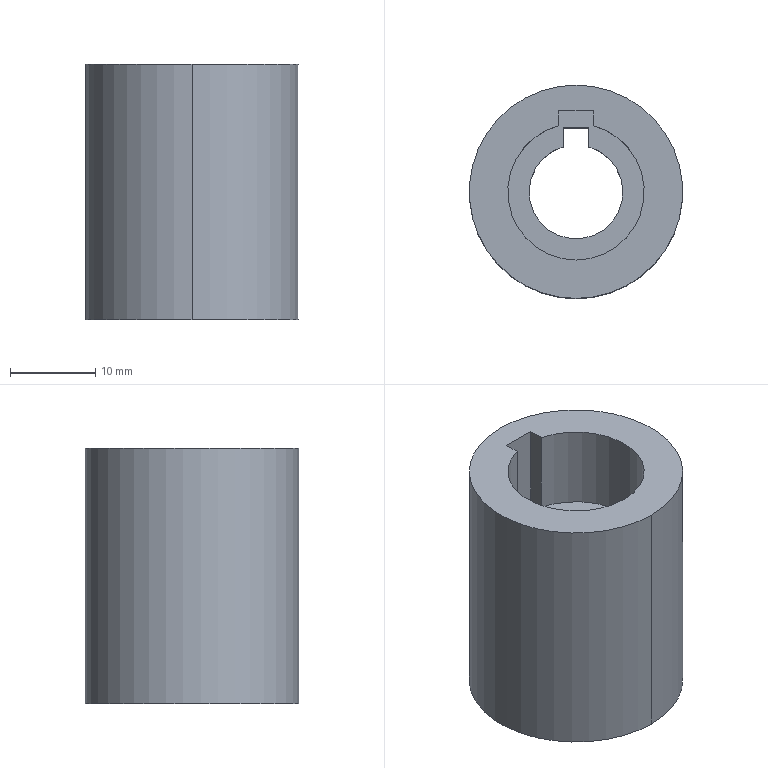Component | SolidWorks | Coupling-1 | 1 solid | 14 faces | box 25 x 25 x 30 mm | volume 10627 mm3 | plane 9 | cylinder 5 | commonest cylinder face diameters 16 x2 25 x2 11 x1
build123d program:
from build123d import *

# Parameters (mm, degrees)
SKETCH1_R               = 12.5
BOSS_EXTRUDE1_DEPTH     = 30
CUT_EXTRUDE1_DEPTH      = 35.821
CUT_EXTRUDE1_DEPTH_BACK = 35.821
SKETCH2_R               = 5
SKETCH3_R               = 8
CUT_EXTRUDE2_DEPTH      = 10
SKETCH4_R               = 5.5
CUT_EXTRUDE3_DEPTH      = 20
SKETCH5_W               = 3
SKETCH5_H               = 4
CUT_EXTRUDE4_DEPTH      = 20
SKETCH6_W               = 4
SKETCH6_H               = 3
CUT_EXTRUDE5_DEPTH      = 10


with BuildPart() as part:
    # Sketch1 → Boss-Extrude1 (new body)
    with BuildSketch(Plane(origin=(0, 0, 0), x_dir=(1, 0, 0), z_dir=(0, 1, 0))):
        with Locations(Location((0, 0, 0), (0, 0, 270))):
            Circle(SKETCH1_R)
    extrude(amount=BOSS_EXTRUDE1_DEPTH)

    # Sketch2 → Cut-Extrude1 (cut, two sides: drawn at the far end of the back side and taken through both)
    with BuildSketch(Plane(origin=(0, 30, 0), x_dir=(1, 0, 0), z_dir=(0, 1, 0)).offset(-CUT_EXTRUDE1_DEPTH_BACK)):
        with Locations(Location((0, 0, 0), (0, 0, 270))):
            Circle(SKETCH2_R)
    extrude(amount=CUT_EXTRUDE1_DEPTH + CUT_EXTRUDE1_DEPTH_BACK, mode=Mode.SUBTRACT)

    # Sketch3 → Cut-Extrude2 (cut)
    with BuildSketch(Plane(origin=(0, 30, 0), x_dir=(1, 0, 0), z_dir=(0, 1, 0))):
        with Locations(Location((0, 0, 0), (0, 0, 270))):
            Circle(SKETCH3_R)
    extrude(amount=-CUT_EXTRUDE2_DEPTH, mode=Mode.SUBTRACT)

    # Sketch4 → Cut-Extrude3 (cut)
    with BuildSketch(Plane.XZ):
        with Locations(Location((0, 0, 0), (0, 0, 270))):
            Circle(SKETCH4_R)
    extrude(amount=-CUT_EXTRUDE3_DEPTH, mode=Mode.SUBTRACT)

    # Sketch5 → Cut-Extrude4 (cut)
    with BuildSketch(Plane.XZ):
        with Locations((0, -5.5)):
            Rectangle(SKETCH5_W, SKETCH5_H)
    extrude(amount=-CUT_EXTRUDE4_DEPTH, mode=Mode.SUBTRACT)

    # Sketch6 → Cut-Extrude5 (cut)
    with BuildSketch(Plane(origin=(0, 30, 0), x_dir=(1, 0, 0), z_dir=(0, 1, 0))):
        with Locations((0, 8)):
            Rectangle(SKETCH6_W, SKETCH6_H)
    extrude(amount=-CUT_EXTRUDE5_DEPTH, mode=Mode.SUBTRACT)


solid = part.part

# Placed as in the assembly
solid = solid.moved(Location((0, -208.707, -673.144), (90, 0, 0)))
STEP:
#1=COLOUR_RGB('',0.7922,0.8196,0.9333);
#2=FILL_AREA_STYLE_COLOUR('',#1);
#3=FILL_AREA_STYLE('',(#2));
#4=SURFACE_STYLE_FILL_AREA(#3);
#5=SURFACE_SIDE_STYLE('',(#4));
#6=SURFACE_STYLE_USAGE(.BOTH.,#5);
#7=PRESENTATION_STYLE_ASSIGNMENT((#6));
#8=CARTESIAN_POINT('',(0.,-8.532,-25.714));
#9=VERTEX_POINT('',#8);
#10=CARTESIAN_POINT('',(0.07874,-7.912,-25.714));
#11=VERTEX_POINT('',#10);
#12=CARTESIAN_POINT('',(-0.,-8.217,-25.714));
#13=DIRECTION('',(0.,0.,1.));
#14=DIRECTION('',(0.,-1.,0.));
#15=AXIS2_PLACEMENT_3D('',#12,#13,#14);
#16=CIRCLE('',#15,0.315);
#17=EDGE_CURVE('',#9,#11,#16,.T.);
#18=ORIENTED_EDGE('',*,*,#17,.F.);
#19=CARTESIAN_POINT('',(0.,-8.532,-25.321));
#20=VERTEX_POINT('',#19);
#21=CARTESIAN_POINT('',(0.,-8.532,-25.714));
#22=DIRECTION('',(0.,0.,1.));
#23=VECTOR('',#22,39.37);
#24=LINE('',#21,#23);
#25=EDGE_CURVE('',#9,#20,#24,.T.);
#26=ORIENTED_EDGE('',*,*,#25,.T.);
#27=CARTESIAN_POINT('',(0.07874,-7.912,-25.321));
#28=VERTEX_POINT('',#27);
#29=CARTESIAN_POINT('',(-0.,-8.217,-25.321));
#30=DIRECTION('',(0.,0.,1.));
#31=DIRECTION('',(0.,-1.,0.));
#32=AXIS2_PLACEMENT_3D('',#29,#30,#31);
#33=CIRCLE('',#32,0.315);
#34=EDGE_CURVE('',#20,#28,#33,.T.);
#35=ORIENTED_EDGE('',*,*,#34,.T.);
#36=CARTESIAN_POINT('',(0.07874,-7.912,-25.714));
#37=DIRECTION('',(-0.,-0.,-1.));
#38=VECTOR('',#37,39.37);
#39=LINE('',#36,#38);
#40=EDGE_CURVE('',#28,#11,#39,.T.);
#41=ORIENTED_EDGE('',*,*,#40,.T.);
#42=EDGE_LOOP('',(#18,#26,#35,#41));
#43=FACE_OUTER_BOUND('',#42,.T.);
#44=CARTESIAN_POINT('',(-0.,-8.217,-25.714));
#45=DIRECTION('',(0.,0.,1.));
#46=DIRECTION('',(0.,-1.,0.));
#47=AXIS2_PLACEMENT_3D('',#44,#45,#46);
#48=CYLINDRICAL_SURFACE('',#47,0.315);
#49=ADVANCED_FACE('',(#43),#48,.F.);
#50=CARTESIAN_POINT('',(0.,-8.709,-25.321));
#51=VERTEX_POINT('',#50);
#52=CARTESIAN_POINT('',(-0.,-7.725,-25.321));
#53=VERTEX_POINT('',#52);
#54=CARTESIAN_POINT('',(-0.,-8.217,-25.321));
#55=DIRECTION('',(0.,0.,1.));
#56=DIRECTION('',(0.,-1.,0.));
#57=AXIS2_PLACEMENT_3D('',#54,#55,#56);
#58=CIRCLE('',#57,0.4921);
#59=EDGE_CURVE('',#51,#53,#58,.T.);
#60=ORIENTED_EDGE('',*,*,#59,.F.);
#61=CARTESIAN_POINT('',(0.,-8.709,-26.502));
#62=VERTEX_POINT('',#61);
#63=CARTESIAN_POINT('',(0.,-8.709,-25.321));
#64=DIRECTION('',(-0.,-0.,-1.));
#65=VECTOR('',#64,39.37);
#66=LINE('',#63,#65);
#67=EDGE_CURVE('',#51,#62,#66,.T.);
#68=ORIENTED_EDGE('',*,*,#67,.T.);
#69=CARTESIAN_POINT('',(-0.,-7.725,-26.502));
#70=VERTEX_POINT('',#69);
#71=CARTESIAN_POINT('',(-0.,-8.217,-26.502));
#72=DIRECTION('',(0.,0.,1.));
#73=DIRECTION('',(0.,-1.,0.));
#74=AXIS2_PLACEMENT_3D('',#71,#72,#73);
#75=CIRCLE('',#74,0.4921);
#76=EDGE_CURVE('',#62,#70,#75,.T.);
#77=ORIENTED_EDGE('',*,*,#76,.T.);
#78=CARTESIAN_POINT('',(-0.,-7.725,-25.321));
#79=DIRECTION('',(-0.,-0.,-1.));
#80=VECTOR('',#79,39.37);
#81=LINE('',#78,#80);
#82=EDGE_CURVE('',#53,#70,#81,.T.);
#83=ORIENTED_EDGE('',*,*,#82,.F.);
#84=EDGE_LOOP('',(#60,#68,#77,#83));
#85=FACE_OUTER_BOUND('',#84,.T.);
#86=CARTESIAN_POINT('',(-0.,-8.217,-25.321));
#87=DIRECTION('',(-0.,-0.,-1.));
#88=DIRECTION('',(-0.,1.,0.));
#89=AXIS2_PLACEMENT_3D('',#86,#87,#88);
#90=CYLINDRICAL_SURFACE('',#89,0.4921);
#91=ADVANCED_FACE('',(#85),#90,.T.);
#92=ORIENTED_EDGE('',*,*,#67,.F.);
#93=CARTESIAN_POINT('',(-0.,-8.217,-25.321));
#94=DIRECTION('',(0.,0.,1.));
#95=DIRECTION('',(0.,-1.,0.));
#96=AXIS2_PLACEMENT_3D('',#93,#94,#95);
#97=CIRCLE('',#96,0.4921);
#98=EDGE_CURVE('',#53,#51,#97,.T.);
#99=ORIENTED_EDGE('',*,*,#98,.F.);
#100=ORIENTED_EDGE('',*,*,#82,.T.);
#101=CARTESIAN_POINT('',(-0.,-8.217,-26.502));
#102=DIRECTION('',(0.,0.,1.));
#103=DIRECTION('',(0.,-1.,0.));
#104=AXIS2_PLACEMENT_3D('',#101,#102,#103);
#105=CIRCLE('',#104,0.4921);
#106=EDGE_CURVE('',#70,#62,#105,.T.);
#107=ORIENTED_EDGE('',*,*,#106,.T.);
#108=EDGE_LOOP('',(#92,#99,#100,#107));
#109=FACE_OUTER_BOUND('',#108,.T.);
#110=CARTESIAN_POINT('',(-0.,-8.217,-25.321));
#111=DIRECTION('',(-0.,-0.,-1.));
#112=DIRECTION('',(-0.,1.,0.));
#113=AXIS2_PLACEMENT_3D('',#110,#111,#112);
#114=CYLINDRICAL_SURFACE('',#113,0.4921);
#115=ADVANCED_FACE('',(#109),#114,.T.);
#116=CARTESIAN_POINT('',(0.07874,-7.843,-25.321));
#117=VERTEX_POINT('',#116);
#118=CARTESIAN_POINT('',(0.07874,-7.961,-25.321));
#119=DIRECTION('',(-0.,1.,-0.));
#120=VECTOR('',#119,39.37);
#121=LINE('',#118,#120);
#122=EDGE_CURVE('',#28,#117,#121,.T.);
#123=ORIENTED_EDGE('',*,*,#122,.F.);
#124=ORIENTED_EDGE('',*,*,#34,.F.);
#125=CARTESIAN_POINT('',(-0.07874,-7.912,-25.321));
#126=VERTEX_POINT('',#125);
#127=CARTESIAN_POINT('',(-0.,-8.217,-25.321));
#128=DIRECTION('',(0.,0.,1.));
#129=DIRECTION('',(0.,-1.,0.));
#130=AXIS2_PLACEMENT_3D('',#127,#128,#129);
#131=CIRCLE('',#130,0.315);
#132=EDGE_CURVE('',#126,#20,#131,.T.);
#133=ORIENTED_EDGE('',*,*,#132,.F.);
#134=CARTESIAN_POINT('',(-0.07874,-7.843,-25.321));
#135=VERTEX_POINT('',#134);
#136=CARTESIAN_POINT('',(-0.07874,-7.961,-25.321));
#137=DIRECTION('',(0.,-1.,0.));
#138=VECTOR('',#137,39.37);
#139=LINE('',#136,#138);
#140=EDGE_CURVE('',#135,#126,#139,.T.);
#141=ORIENTED_EDGE('',*,*,#140,.F.);
#142=CARTESIAN_POINT('',(-0.07874,-7.843,-25.321));
#143=DIRECTION('',(-1.,-0.,0.));
#144=VECTOR('',#143,39.37);
#145=LINE('',#142,#144);
#146=EDGE_CURVE('',#117,#135,#145,.T.);
#147=ORIENTED_EDGE('',*,*,#146,.F.);
#148=EDGE_LOOP('',(#123,#124,#133,#141,#147));
#149=FACE_BOUND('',#148,.T.);
#150=ORIENTED_EDGE('',*,*,#98,.T.);
#151=ORIENTED_EDGE('',*,*,#59,.T.);
#152=EDGE_LOOP('',(#150,#151));
#153=FACE_OUTER_BOUND('',#152,.T.);
#154=CARTESIAN_POINT('',(-0.,-8.217,-25.321));
#155=DIRECTION('',(0.,0.,1.));
#156=DIRECTION('',(0.,-1.,0.));
#157=AXIS2_PLACEMENT_3D('',#154,#155,#156);
#158=PLANE('',#157);
#159=ADVANCED_FACE('',(#149,#153),#158,.T.);
#160=CARTESIAN_POINT('',(-0.05906,-7.922,-26.502));
#161=VERTEX_POINT('',#160);
#162=CARTESIAN_POINT('',(0.05906,-7.922,-26.502));
#163=VERTEX_POINT('',#162);
#164=CARTESIAN_POINT('',(0.05906,-7.922,-26.502));
#165=DIRECTION('',(1.,0.,-0.));
#166=VECTOR('',#165,39.37);
#167=LINE('',#164,#166);
#168=EDGE_CURVE('',#161,#163,#167,.T.);
#169=ORIENTED_EDGE('',*,*,#168,.F.);
#170=CARTESIAN_POINT('',(-0.05906,-8.009,-26.502));
#171=VERTEX_POINT('',#170);
#172=CARTESIAN_POINT('',(-0.05906,-8.079,-26.502));
#173=DIRECTION('',(-0.,1.,-0.));
#174=VECTOR('',#173,39.37);
#175=LINE('',#172,#174);
#176=EDGE_CURVE('',#171,#161,#175,.T.);
#177=ORIENTED_EDGE('',*,*,#176,.F.);
#178=CARTESIAN_POINT('',(0.05906,-8.009,-26.502));
#179=VERTEX_POINT('',#178);
#180=CARTESIAN_POINT('',(-0.,-8.217,-26.502));
#181=DIRECTION('',(-0.,-0.,-1.));
#182=DIRECTION('',(-0.,1.,0.));
#183=AXIS2_PLACEMENT_3D('',#180,#181,#182);
#184=CIRCLE('',#183,0.2165);
#185=EDGE_CURVE('',#179,#171,#184,.T.);
#186=ORIENTED_EDGE('',*,*,#185,.F.);
#187=CARTESIAN_POINT('',(0.05906,-8.079,-26.502));
#188=DIRECTION('',(0.,-1.,0.));
#189=VECTOR('',#188,39.37);
#190=LINE('',#187,#189);
#191=EDGE_CURVE('',#163,#179,#190,.T.);
#192=ORIENTED_EDGE('',*,*,#191,.F.);
#193=EDGE_LOOP('',(#169,#177,#186,#192));
#194=FACE_BOUND('',#193,.T.);
#195=ORIENTED_EDGE('',*,*,#106,.F.);
#196=ORIENTED_EDGE('',*,*,#76,.F.);
#197=EDGE_LOOP('',(#195,#196));
#198=FACE_OUTER_BOUND('',#197,.T.);
#199=CARTESIAN_POINT('',(-0.,-8.217,-26.502));
#200=DIRECTION('',(0.,0.,1.));
#201=DIRECTION('',(0.,-1.,0.));
#202=AXIS2_PLACEMENT_3D('',#199,#200,#201);
#203=PLANE('',#202);
#204=ADVANCED_FACE('',(#194,#198),#203,.F.);
#205=CARTESIAN_POINT('',(-0.07874,-7.912,-25.714));
#206=VERTEX_POINT('',#205);
#207=CARTESIAN_POINT('',(-0.,-8.217,-25.714));
#208=DIRECTION('',(0.,0.,1.));
#209=DIRECTION('',(0.,-1.,0.));
#210=AXIS2_PLACEMENT_3D('',#207,#208,#209);
#211=CIRCLE('',#210,0.315);
#212=EDGE_CURVE('',#206,#9,#211,.T.);
#213=ORIENTED_EDGE('',*,*,#212,.T.);
#214=ORIENTED_EDGE('',*,*,#17,.T.);
#215=CARTESIAN_POINT('',(0.07874,-7.843,-25.714));
#216=VERTEX_POINT('',#215);
#217=CARTESIAN_POINT('',(0.07874,-7.961,-25.714));
#218=DIRECTION('',(-0.,1.,-0.));
#219=VECTOR('',#218,39.37);
#220=LINE('',#217,#219);
#221=EDGE_CURVE('',#11,#216,#220,.T.);
#222=ORIENTED_EDGE('',*,*,#221,.T.);
#223=CARTESIAN_POINT('',(-0.07874,-7.843,-25.714));
#224=VERTEX_POINT('',#223);
#225=CARTESIAN_POINT('',(-0.07874,-7.843,-25.714));
#226=DIRECTION('',(-1.,-0.,0.));
#227=VECTOR('',#226,39.37);
#228=LINE('',#225,#227);
#229=EDGE_CURVE('',#216,#224,#228,.T.);
#230=ORIENTED_EDGE('',*,*,#229,.T.);
#231=CARTESIAN_POINT('',(-0.07874,-7.961,-25.714));
#232=DIRECTION('',(0.,-1.,0.));
#233=VECTOR('',#232,39.37);
#234=LINE('',#231,#233);
#235=EDGE_CURVE('',#224,#206,#234,.T.);
#236=ORIENTED_EDGE('',*,*,#235,.T.);
#237=EDGE_LOOP('',(#213,#214,#222,#230,#236));
#238=FACE_OUTER_BOUND('',#237,.T.);
#239=CARTESIAN_POINT('',(-0.05906,-8.009,-25.714));
#240=VERTEX_POINT('',#239);
#241=CARTESIAN_POINT('',(-0.05906,-7.922,-25.714));
#242=VERTEX_POINT('',#241);
#243=CARTESIAN_POINT('',(-0.05906,-8.079,-25.714));
#244=DIRECTION('',(-0.,1.,-0.));
#245=VECTOR('',#244,39.37);
#246=LINE('',#243,#245);
#247=EDGE_CURVE('',#240,#242,#246,.T.);
#248=ORIENTED_EDGE('',*,*,#247,.T.);
#249=CARTESIAN_POINT('',(0.05906,-7.922,-25.714));
#250=VERTEX_POINT('',#249);
#251=CARTESIAN_POINT('',(0.05906,-7.922,-25.714));
#252=DIRECTION('',(1.,0.,-0.));
#253=VECTOR('',#252,39.37);
#254=LINE('',#251,#253);
#255=EDGE_CURVE('',#242,#250,#254,.T.);
#256=ORIENTED_EDGE('',*,*,#255,.T.);
#257=CARTESIAN_POINT('',(0.05906,-8.009,-25.714));
#258=VERTEX_POINT('',#257);
#259=CARTESIAN_POINT('',(0.05906,-8.079,-25.714));
#260=DIRECTION('',(0.,-1.,0.));
#261=VECTOR('',#260,39.37);
#262=LINE('',#259,#261);
#263=EDGE_CURVE('',#250,#258,#262,.T.);
#264=ORIENTED_EDGE('',*,*,#263,.T.);
#265=CARTESIAN_POINT('',(-0.,-8.217,-25.714));
#266=DIRECTION('',(-0.,-0.,-1.));
#267=DIRECTION('',(-0.,1.,0.));
#268=AXIS2_PLACEMENT_3D('',#265,#266,#267);
#269=CIRCLE('',#268,0.2165);
#270=EDGE_CURVE('',#258,#240,#269,.T.);
#271=ORIENTED_EDGE('',*,*,#270,.T.);
#272=EDGE_LOOP('',(#248,#256,#264,#271));
#273=FACE_BOUND('',#272,.T.);
#274=CARTESIAN_POINT('',(-0.,-8.217,-25.714));
#275=DIRECTION('',(0.,0.,1.));
#276=DIRECTION('',(0.,-1.,0.));
#277=AXIS2_PLACEMENT_3D('',#274,#275,#276);
#278=PLANE('',#277);
#279=ADVANCED_FACE('',(#238,#273),#278,.T.);
#280=ORIENTED_EDGE('',*,*,#25,.F.);
#281=ORIENTED_EDGE('',*,*,#212,.F.);
#282=CARTESIAN_POINT('',(-0.07874,-7.912,-25.714));
#283=DIRECTION('',(0.,0.,1.));
#284=VECTOR('',#283,39.37);
#285=LINE('',#282,#284);
#286=EDGE_CURVE('',#206,#126,#285,.T.);
#287=ORIENTED_EDGE('',*,*,#286,.T.);
#288=ORIENTED_EDGE('',*,*,#132,.T.);
#289=EDGE_LOOP('',(#280,#281,#287,#288));
#290=FACE_OUTER_BOUND('',#289,.T.);
#291=CARTESIAN_POINT('',(-0.,-8.217,-25.714));
#292=DIRECTION('',(0.,0.,1.));
#293=DIRECTION('',(0.,-1.,0.));
#294=AXIS2_PLACEMENT_3D('',#291,#292,#293);
#295=CYLINDRICAL_SURFACE('',#294,0.315);
#296=ADVANCED_FACE('',(#290),#295,.F.);
#297=ORIENTED_EDGE('',*,*,#185,.T.);
#298=CARTESIAN_POINT('',(-0.05906,-8.009,-25.714));
#299=DIRECTION('',(0.,0.,1.));
#300=VECTOR('',#299,39.37);
#301=LINE('',#298,#300);
#302=EDGE_CURVE('',#171,#240,#301,.T.);
#303=ORIENTED_EDGE('',*,*,#302,.T.);
#304=ORIENTED_EDGE('',*,*,#270,.F.);
#305=CARTESIAN_POINT('',(0.05906,-8.009,-25.714));
#306=DIRECTION('',(-0.,-0.,-1.));
#307=VECTOR('',#306,39.37);
#308=LINE('',#305,#307);
#309=EDGE_CURVE('',#258,#179,#308,.T.);
#310=ORIENTED_EDGE('',*,*,#309,.T.);
#311=EDGE_LOOP('',(#297,#303,#304,#310));
#312=FACE_OUTER_BOUND('',#311,.T.);
#313=CARTESIAN_POINT('',(-0.,-8.217,-25.714));
#314=DIRECTION('',(-0.,-0.,-1.));
#315=DIRECTION('',(-0.,1.,0.));
#316=AXIS2_PLACEMENT_3D('',#313,#314,#315);
#317=CYLINDRICAL_SURFACE('',#316,0.2165);
#318=ADVANCED_FACE('',(#312),#317,.F.);
#319=ORIENTED_EDGE('',*,*,#176,.T.);
#320=CARTESIAN_POINT('',(-0.05906,-7.922,-25.714));
#321=DIRECTION('',(-0.,-0.,-1.));
#322=VECTOR('',#321,39.37);
#323=LINE('',#320,#322);
#324=EDGE_CURVE('',#242,#161,#323,.T.);
#325=ORIENTED_EDGE('',*,*,#324,.F.);
#326=ORIENTED_EDGE('',*,*,#247,.F.);
#327=ORIENTED_EDGE('',*,*,#302,.F.);
#328=EDGE_LOOP('',(#319,#325,#326,#327));
#329=FACE_OUTER_BOUND('',#328,.T.);
#330=CARTESIAN_POINT('',(-0.05906,-8.079,-25.714));
#331=DIRECTION('',(-1.,-0.,0.));
#332=DIRECTION('',(0.,-1.,0.));
#333=AXIS2_PLACEMENT_3D('',#330,#331,#332);
#334=PLANE('',#333);
#335=ADVANCED_FACE('',(#329),#334,.F.);
#336=ORIENTED_EDGE('',*,*,#263,.F.);
#337=CARTESIAN_POINT('',(0.05906,-7.922,-25.714));
#338=DIRECTION('',(-0.,-0.,-1.));
#339=VECTOR('',#338,39.37);
#340=LINE('',#337,#339);
#341=EDGE_CURVE('',#250,#163,#340,.T.);
#342=ORIENTED_EDGE('',*,*,#341,.T.);
#343=ORIENTED_EDGE('',*,*,#191,.T.);
#344=ORIENTED_EDGE('',*,*,#309,.F.);
#345=EDGE_LOOP('',(#336,#342,#343,#344));
#346=FACE_OUTER_BOUND('',#345,.T.);
#347=CARTESIAN_POINT('',(0.05906,-8.079,-25.714));
#348=DIRECTION('',(1.,0.,-0.));
#349=DIRECTION('',(-0.,1.,-0.));
#350=AXIS2_PLACEMENT_3D('',#347,#348,#349);
#351=PLANE('',#350);
#352=ADVANCED_FACE('',(#346),#351,.F.);
#353=ORIENTED_EDGE('',*,*,#168,.T.);
#354=ORIENTED_EDGE('',*,*,#341,.F.);
#355=ORIENTED_EDGE('',*,*,#255,.F.);
#356=ORIENTED_EDGE('',*,*,#324,.T.);
#357=EDGE_LOOP('',(#353,#354,#355,#356));
#358=FACE_OUTER_BOUND('',#357,.T.);
#359=CARTESIAN_POINT('',(0.05906,-7.922,-25.714));
#360=DIRECTION('',(-0.,1.,-0.));
#361=DIRECTION('',(-1.,-0.,0.));
#362=AXIS2_PLACEMENT_3D('',#359,#360,#361);
#363=PLANE('',#362);
#364=ADVANCED_FACE('',(#358),#363,.F.);
#365=ORIENTED_EDGE('',*,*,#122,.T.);
#366=CARTESIAN_POINT('',(0.07874,-7.843,-25.714));
#367=DIRECTION('',(0.,0.,1.));
#368=VECTOR('',#367,39.37);
#369=LINE('',#366,#368);
#370=EDGE_CURVE('',#216,#117,#369,.T.);
#371=ORIENTED_EDGE('',*,*,#370,.F.);
#372=ORIENTED_EDGE('',*,*,#221,.F.);
#373=ORIENTED_EDGE('',*,*,#40,.F.);
#374=EDGE_LOOP('',(#365,#371,#372,#373));
#375=FACE_OUTER_BOUND('',#374,.T.);
#376=CARTESIAN_POINT('',(0.07874,-7.961,-25.714));
#377=DIRECTION('',(1.,0.,-0.));
#378=DIRECTION('',(-0.,1.,-0.));
#379=AXIS2_PLACEMENT_3D('',#376,#377,#378);
#380=PLANE('',#379);
#381=ADVANCED_FACE('',(#375),#380,.F.);
#382=ORIENTED_EDGE('',*,*,#235,.F.);
#383=CARTESIAN_POINT('',(-0.07874,-7.843,-25.714));
#384=DIRECTION('',(0.,0.,1.));
#385=VECTOR('',#384,39.37);
#386=LINE('',#383,#385);
#387=EDGE_CURVE('',#224,#135,#386,.T.);
#388=ORIENTED_EDGE('',*,*,#387,.T.);
#389=ORIENTED_EDGE('',*,*,#140,.T.);
#390=ORIENTED_EDGE('',*,*,#286,.F.);
#391=EDGE_LOOP('',(#382,#388,#389,#390));
#392=FACE_OUTER_BOUND('',#391,.T.);
#393=CARTESIAN_POINT('',(-0.07874,-7.961,-25.714));
#394=DIRECTION('',(-1.,-0.,0.));
#395=DIRECTION('',(0.,-1.,0.));
#396=AXIS2_PLACEMENT_3D('',#393,#394,#395);
#397=PLANE('',#396);
#398=ADVANCED_FACE('',(#392),#397,.F.);
#399=ORIENTED_EDGE('',*,*,#146,.T.);
#400=ORIENTED_EDGE('',*,*,#387,.F.);
#401=ORIENTED_EDGE('',*,*,#229,.F.);
#402=ORIENTED_EDGE('',*,*,#370,.T.);
#403=EDGE_LOOP('',(#399,#400,#401,#402));
#404=FACE_OUTER_BOUND('',#403,.T.);
#405=CARTESIAN_POINT('',(-0.07874,-7.843,-25.714));
#406=DIRECTION('',(-0.,1.,-0.));
#407=DIRECTION('',(-1.,-0.,0.));
#408=AXIS2_PLACEMENT_3D('',#405,#406,#407);
#409=PLANE('',#408);
#410=ADVANCED_FACE('',(#404),#409,.F.);
#411=CLOSED_SHELL('',(#49,#91,#115,#159,#204,#279,#296,#318,#335,#352,#364,#381,#398,#410));
#412=MANIFOLD_SOLID_BREP('',#411);
#413=STYLED_ITEM('',(#7),#412);
#414=PRESENTATION_LAYER_ASSIGNMENT('','',(#413));
#415=(LENGTH_UNIT()NAMED_UNIT(*)SI_UNIT($,.METRE.));
#416=LENGTH_MEASURE_WITH_UNIT(LENGTH_MEASURE(0.0254),#415);
#417=DIMENSIONAL_EXPONENTS(1.,0.,0.,0.,0.,0.,0.);
#418=(CONVERSION_BASED_UNIT('',#416)LENGTH_UNIT()NAMED_UNIT(#417));
#419=UNCERTAINTY_MEASURE_WITH_UNIT(LENGTH_MEASURE(0.00001),#418,'','');
#420=(NAMED_UNIT(*)PLANE_ANGLE_UNIT()SI_UNIT($,.RADIAN.));
#421=(NAMED_UNIT(*)SI_UNIT($,.STERADIAN.)SOLID_ANGLE_UNIT());
#422=(GEOMETRIC_REPRESENTATION_CONTEXT(3)GLOBAL_UNCERTAINTY_ASSIGNED_CONTEXT((#419))GLOBAL_UNIT_ASSIGNED_CONTEXT((#418,#420,#421))REPRESENTATION_CONTEXT('',''));
#423=MECHANICAL_DESIGN_GEOMETRIC_PRESENTATION_REPRESENTATION('',(#413),#422);
#424=CARTESIAN_POINT('',(0.,0.,0.));
#425=DIRECTION('',(0.,0.,1.));
#426=DIRECTION('',(1.,0.,0.));
#427=AXIS2_PLACEMENT_3D('',#424,#425,#426);
#428=(LENGTH_UNIT()NAMED_UNIT(*)SI_UNIT($,.METRE.));
#429=LENGTH_MEASURE_WITH_UNIT(LENGTH_MEASURE(0.0254),#428);
#430=DIMENSIONAL_EXPONENTS(1.,0.,0.,0.,0.,0.,0.);
#431=(CONVERSION_BASED_UNIT('',#429)LENGTH_UNIT()NAMED_UNIT(#430));
#432=UNCERTAINTY_MEASURE_WITH_UNIT(LENGTH_MEASURE(0.00001),#431,'','');
#433=(NAMED_UNIT(*)PLANE_ANGLE_UNIT()SI_UNIT($,.RADIAN.));
#434=(NAMED_UNIT(*)SI_UNIT($,.STERADIAN.)SOLID_ANGLE_UNIT());
#435=(GEOMETRIC_REPRESENTATION_CONTEXT(3)GLOBAL_UNCERTAINTY_ASSIGNED_CONTEXT((#432))GLOBAL_UNIT_ASSIGNED_CONTEXT((#431,#433,#434))REPRESENTATION_CONTEXT('',''));
#436=ADVANCED_BREP_SHAPE_REPRESENTATION('',(#412,#427),#435);